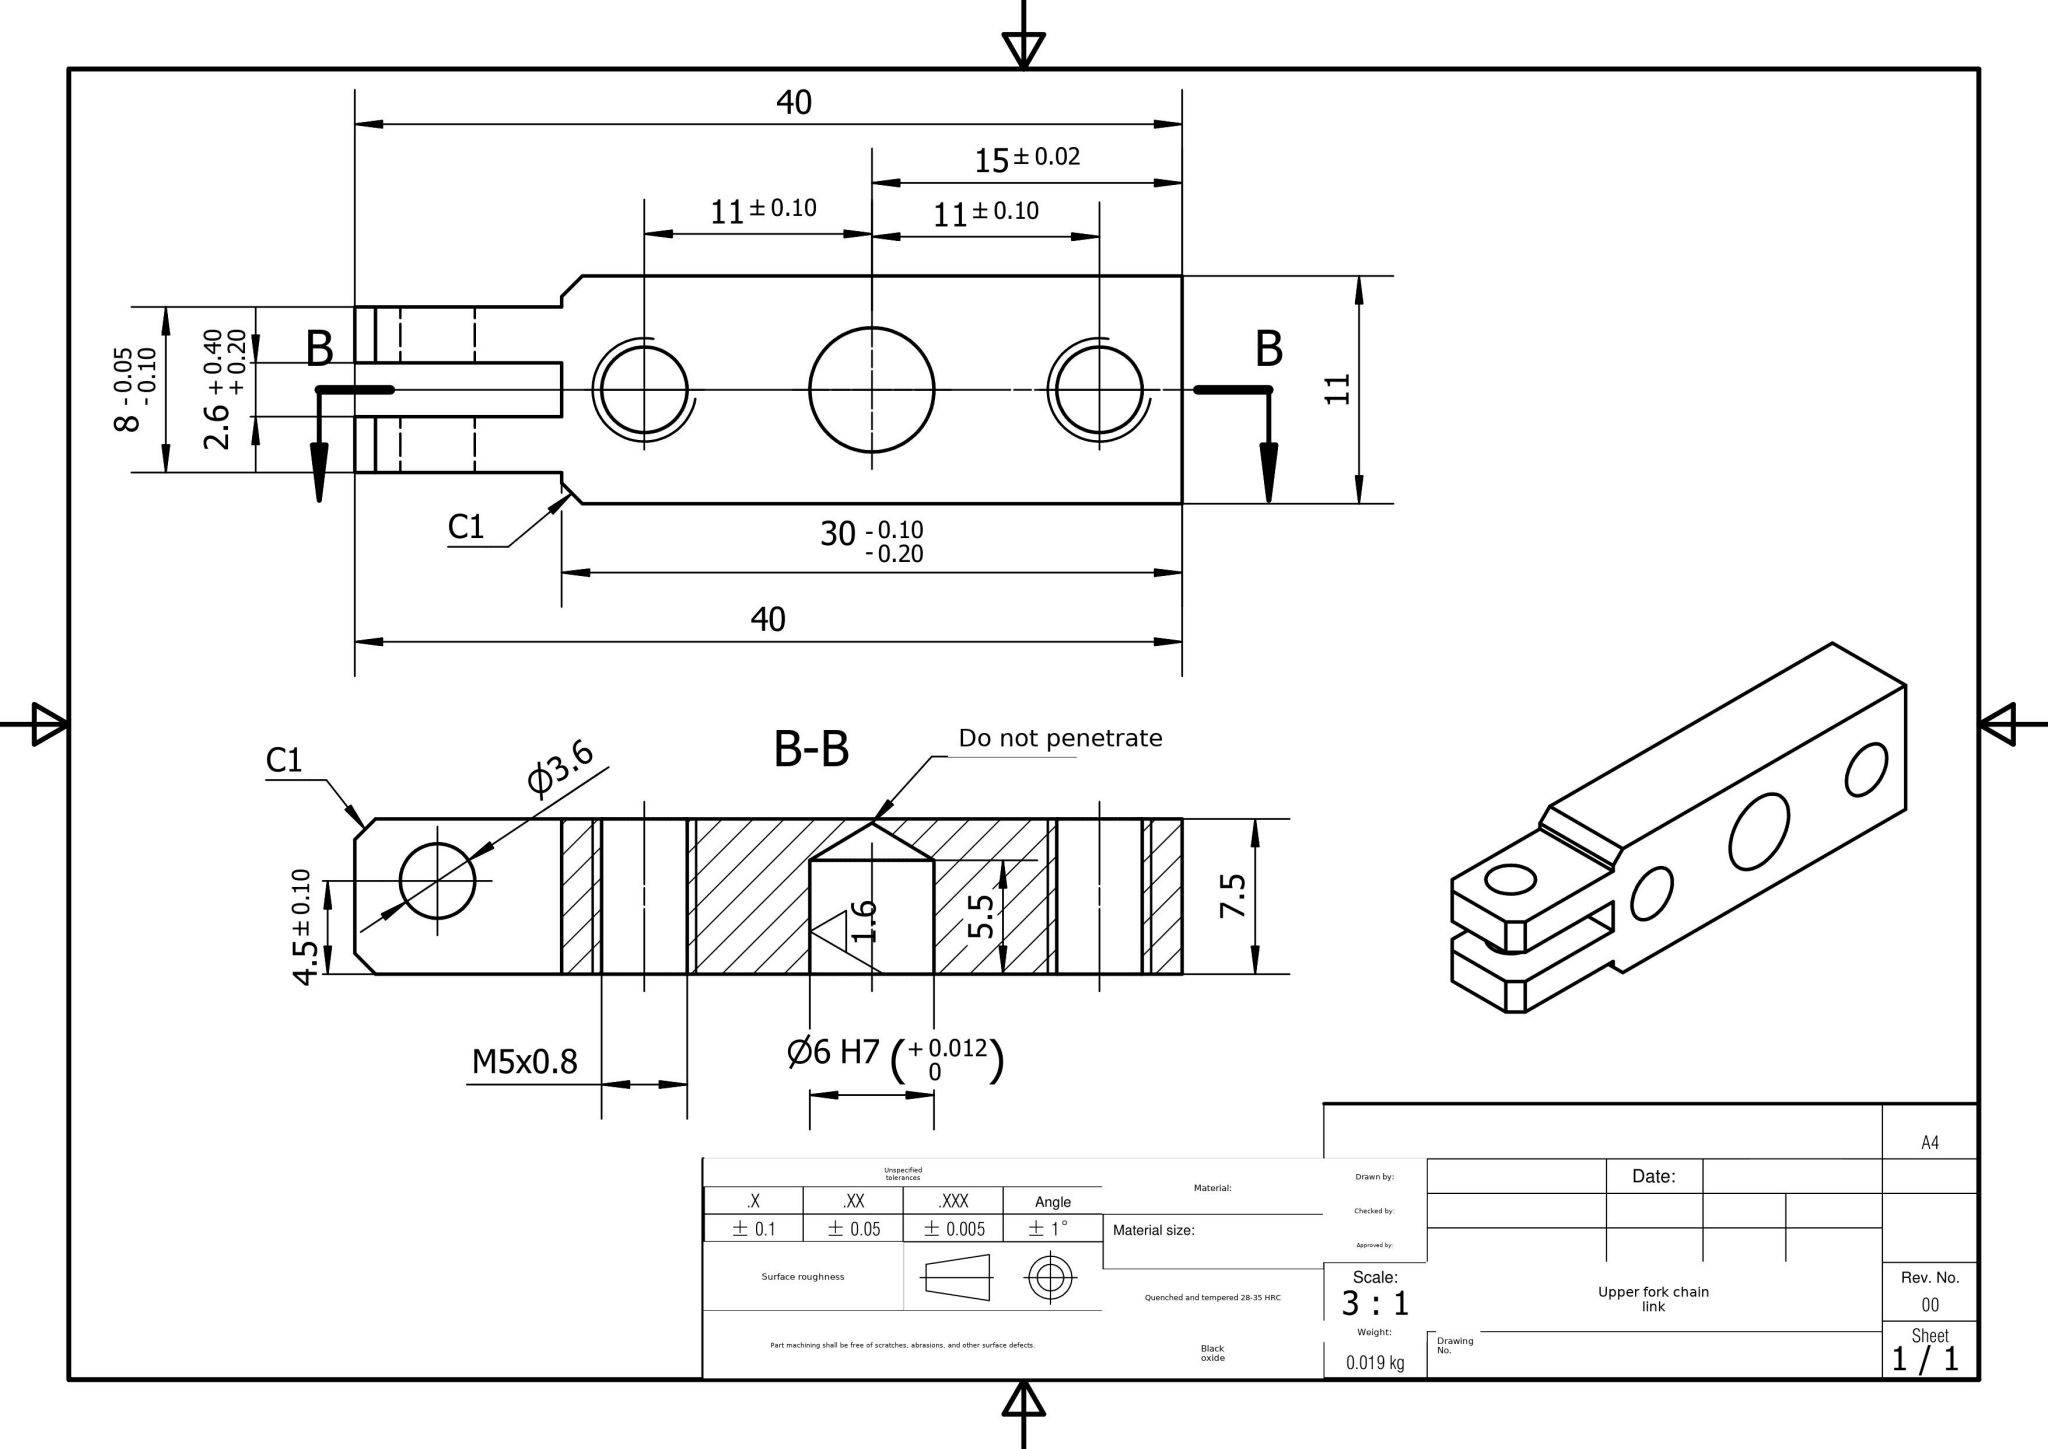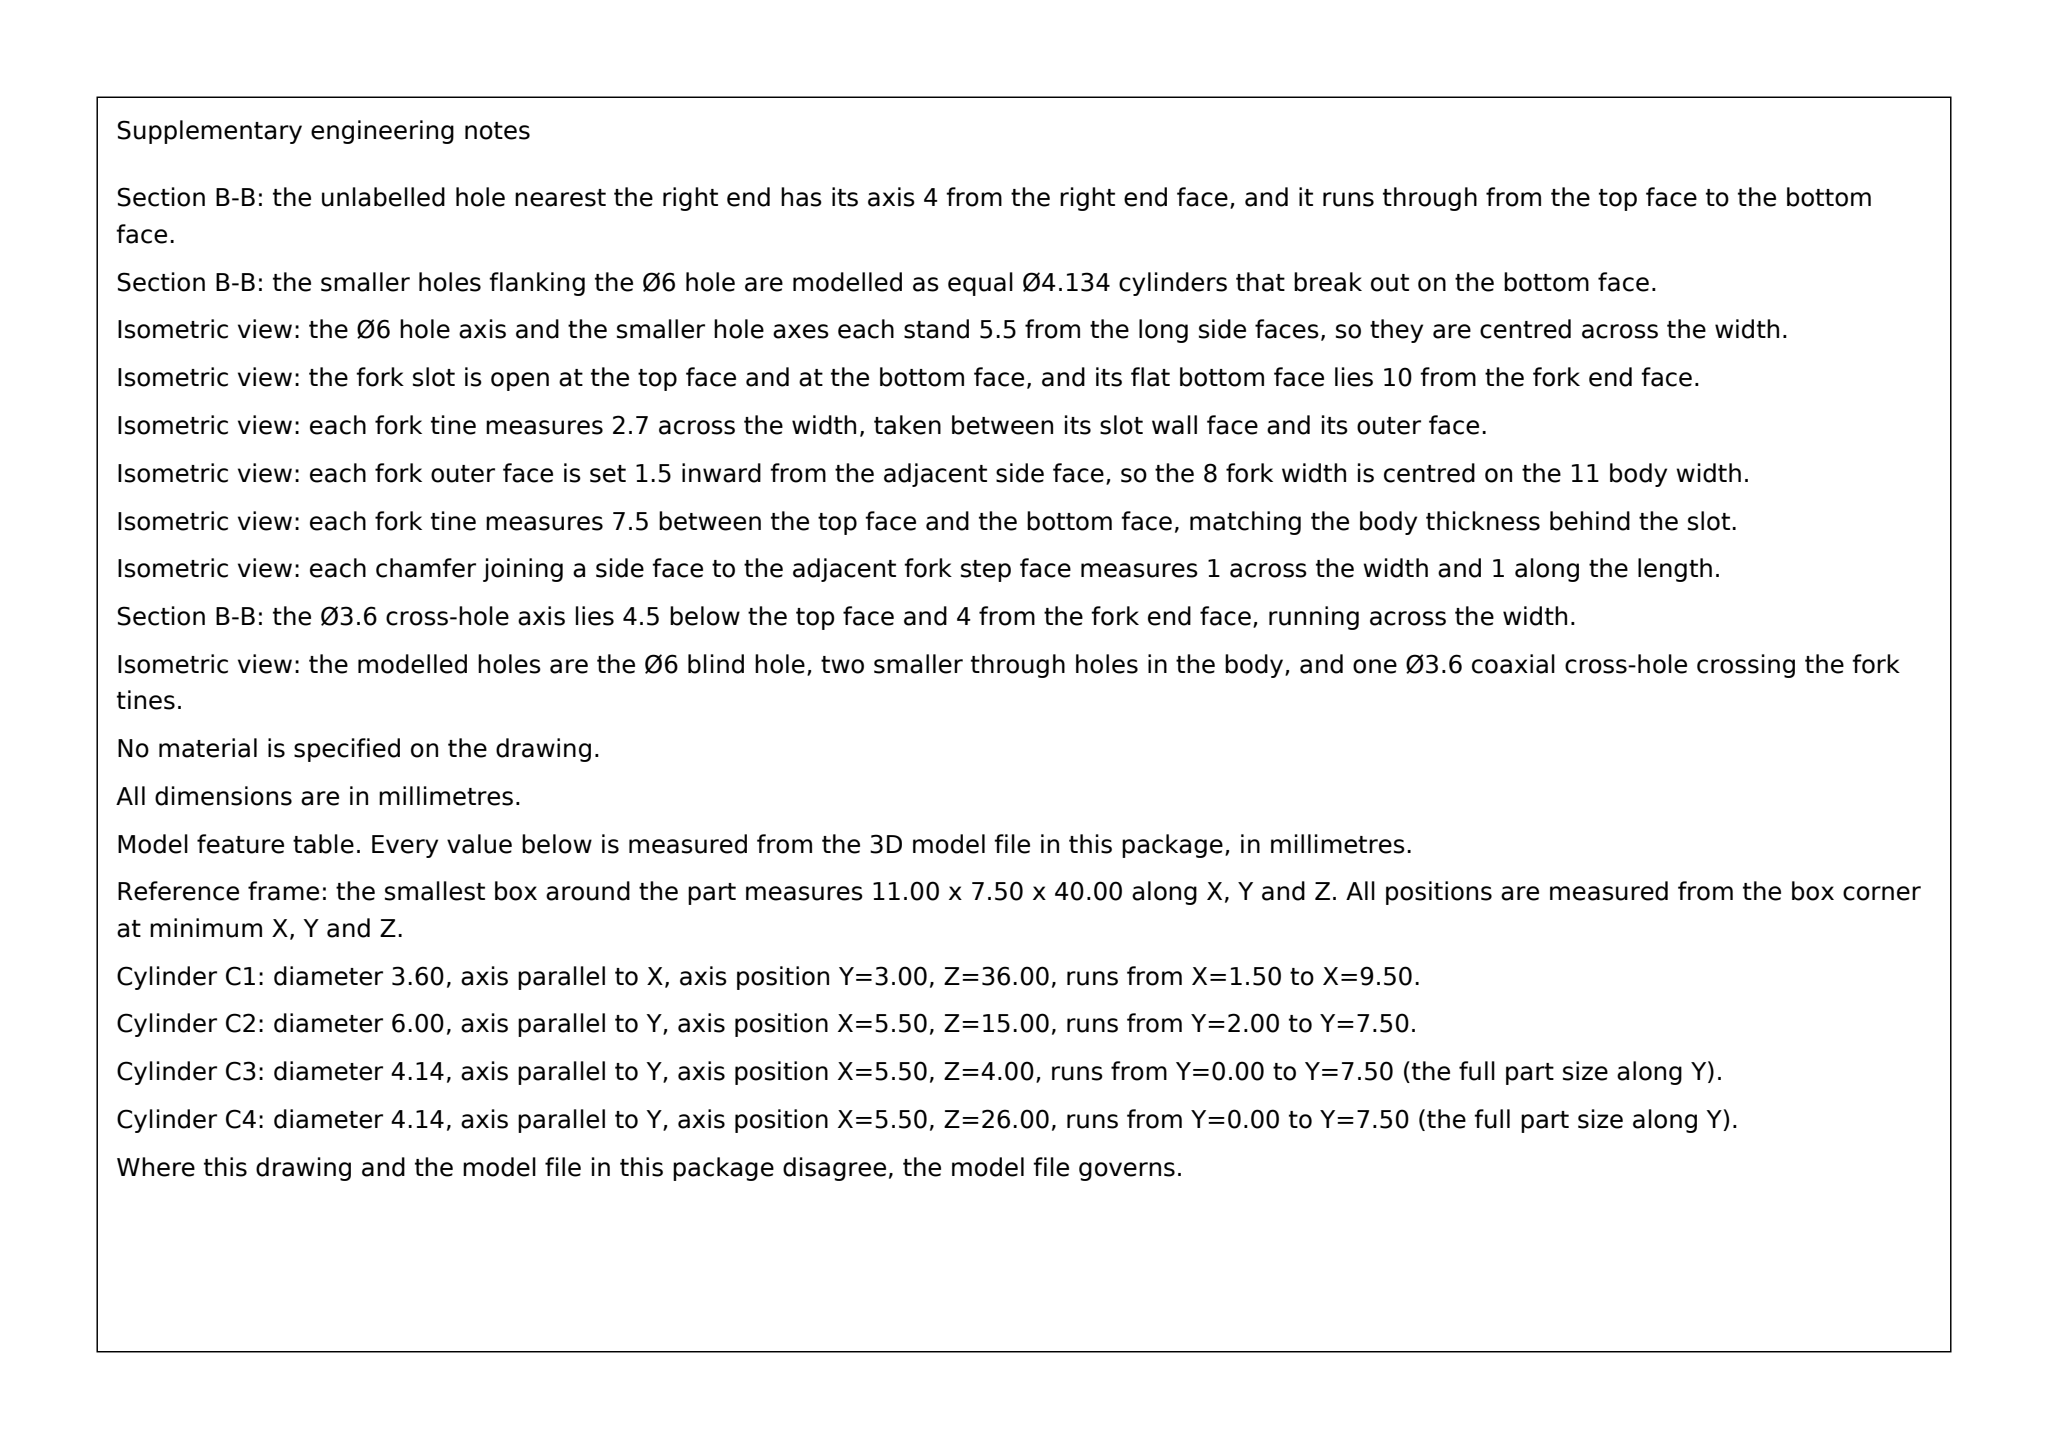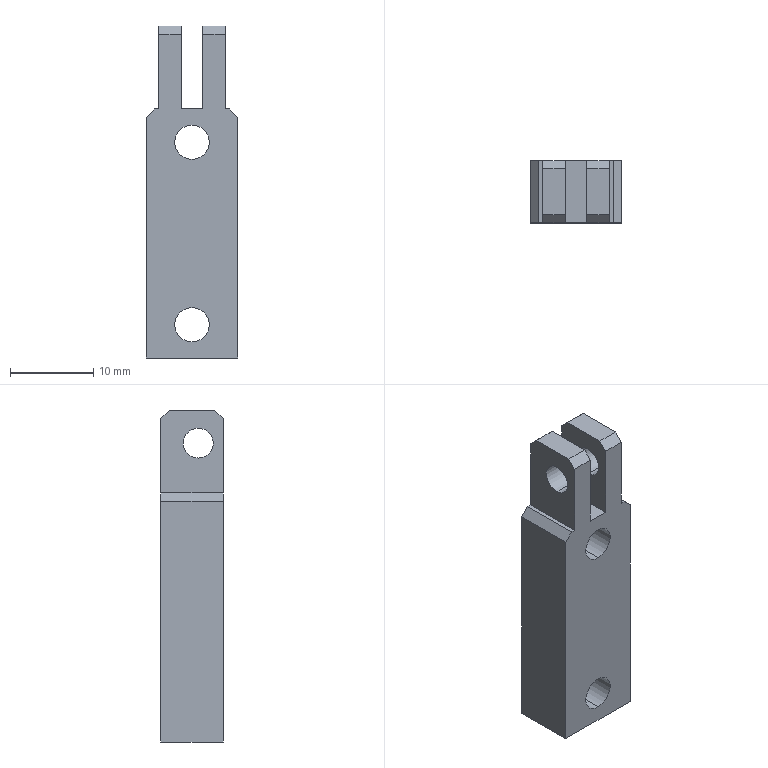Part | SolidWorks | mm | 1 solid | 32 faces | box 11 x 7.5 x 40 mm | volume 2438 mm3 | plane 20 | cylinder 10 | cone 2 | commonest cylinder face diameters 4.134 x4 3.6 x4 6 x2
Drawing notes:
Ø3.6 CROSS HOLE C/L 4 FROM FORK END FACE | from the solid: cyl dia 3.6 axis x at z=36.0; bbox z length 40.0 -> 40-36=4 from fork end face